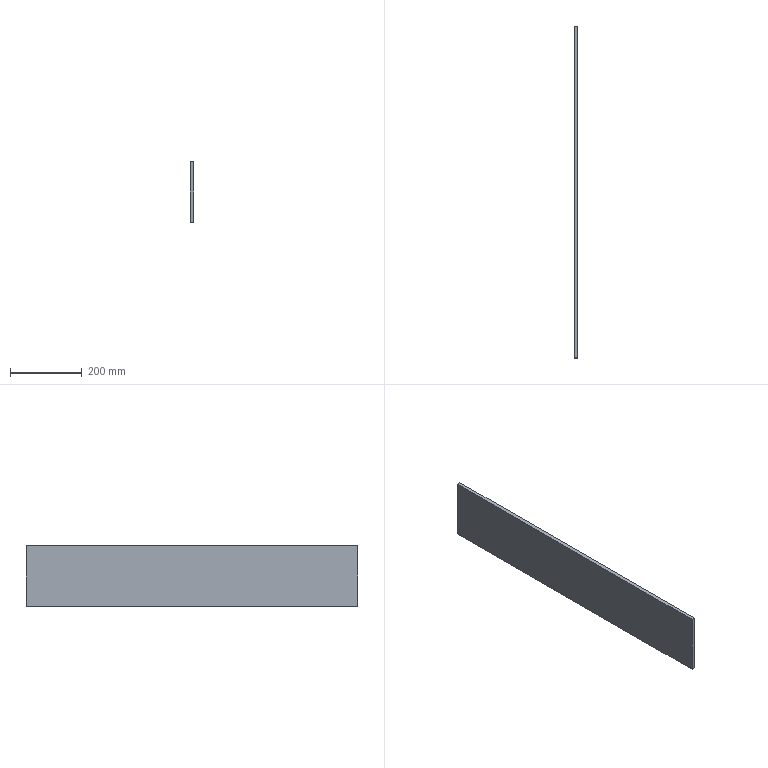Component | SolidWorks | SolderBoxFixingBracketOne-2 | 1 solid | 6 faces | box 10 x 925 x 170 mm | volume 1572500 mm3 | plane 6 | material Plain Carbon Steel
build123d program:
from build123d import *

# Parameters (mm, degrees)
SKETCH1_W           = 925
SKETCH1_H           = 170
BOSS_EXTRUDE1_DEPTH = 10


with BuildPart() as part:
    # Sketch1 → Boss-Extrude1 (new body)
    with BuildSketch(Plane.XY):
        Rectangle(SKETCH1_W, SKETCH1_H)
    extrude(amount=BOSS_EXTRUDE1_DEPTH)


solid = part.part

# Placed as in the assembly
solid = solid.moved(Location((-762.135, 81.593, 1078.102), (90, -90, 0)))
STEP:
#1=COLOUR_RGB('',0.7922,0.8196,0.9333);
#2=FILL_AREA_STYLE_COLOUR('',#1);
#3=FILL_AREA_STYLE('',(#2));
#4=SURFACE_STYLE_FILL_AREA(#3);
#5=SURFACE_SIDE_STYLE('',(#4));
#6=SURFACE_STYLE_USAGE(.BOTH.,#5);
#7=PRESENTATION_STYLE_ASSIGNMENT((#6));
#8=CARTESIAN_POINT('',(-30.399,-14.996,45.791));
#9=VERTEX_POINT('',#8);
#10=CARTESIAN_POINT('',(-30.399,-14.996,39.099));
#11=VERTEX_POINT('',#10);
#12=CARTESIAN_POINT('',(-30.399,-14.996,39.099));
#13=DIRECTION('',(-0.,0.,-1.));
#14=VECTOR('',#13,39.37);
#15=LINE('',#12,#14);
#16=EDGE_CURVE('',#9,#11,#15,.T.);
#17=ORIENTED_EDGE('',*,*,#16,.T.);
#18=CARTESIAN_POINT('',(-30.005,-14.996,39.099));
#19=VERTEX_POINT('',#18);
#20=CARTESIAN_POINT('',(-30.005,-14.996,39.099));
#21=DIRECTION('',(-1.,-0.,0.));
#22=VECTOR('',#21,39.37);
#23=LINE('',#20,#22);
#24=EDGE_CURVE('',#19,#11,#23,.T.);
#25=ORIENTED_EDGE('',*,*,#24,.F.);
#26=CARTESIAN_POINT('',(-30.005,-14.996,45.791));
#27=VERTEX_POINT('',#26);
#28=CARTESIAN_POINT('',(-30.005,-14.996,39.099));
#29=DIRECTION('',(-0.,0.,-1.));
#30=VECTOR('',#29,39.37);
#31=LINE('',#28,#30);
#32=EDGE_CURVE('',#27,#19,#31,.T.);
#33=ORIENTED_EDGE('',*,*,#32,.F.);
#34=CARTESIAN_POINT('',(-30.005,-14.996,45.791));
#35=DIRECTION('',(-1.,-0.,0.));
#36=VECTOR('',#35,39.37);
#37=LINE('',#34,#36);
#38=EDGE_CURVE('',#27,#9,#37,.T.);
#39=ORIENTED_EDGE('',*,*,#38,.T.);
#40=EDGE_LOOP('',(#17,#25,#33,#39));
#41=FACE_OUTER_BOUND('',#40,.T.);
#42=CARTESIAN_POINT('',(-30.005,-14.996,39.099));
#43=DIRECTION('',(-0.,1.,0.));
#44=DIRECTION('',(-1.,-0.,0.));
#45=AXIS2_PLACEMENT_3D('',#42,#43,#44);
#46=PLANE('',#45);
#47=ADVANCED_FACE('',(#41),#46,.F.);
#48=CARTESIAN_POINT('',(-30.399,21.421,39.099));
#49=VERTEX_POINT('',#48);
#50=CARTESIAN_POINT('',(-30.399,21.421,39.099));
#51=DIRECTION('',(-0.,1.,0.));
#52=VECTOR('',#51,39.37);
#53=LINE('',#50,#52);
#54=EDGE_CURVE('',#11,#49,#53,.T.);
#55=ORIENTED_EDGE('',*,*,#54,.T.);
#56=CARTESIAN_POINT('',(-30.005,21.421,39.099));
#57=VERTEX_POINT('',#56);
#58=CARTESIAN_POINT('',(-30.005,21.421,39.099));
#59=DIRECTION('',(-1.,-0.,0.));
#60=VECTOR('',#59,39.37);
#61=LINE('',#58,#60);
#62=EDGE_CURVE('',#57,#49,#61,.T.);
#63=ORIENTED_EDGE('',*,*,#62,.F.);
#64=CARTESIAN_POINT('',(-30.005,21.421,39.099));
#65=DIRECTION('',(-0.,1.,0.));
#66=VECTOR('',#65,39.37);
#67=LINE('',#64,#66);
#68=EDGE_CURVE('',#19,#57,#67,.T.);
#69=ORIENTED_EDGE('',*,*,#68,.F.);
#70=ORIENTED_EDGE('',*,*,#24,.T.);
#71=EDGE_LOOP('',(#55,#63,#69,#70));
#72=FACE_OUTER_BOUND('',#71,.T.);
#73=CARTESIAN_POINT('',(-30.005,21.421,39.099));
#74=DIRECTION('',(0.,-0.,1.));
#75=DIRECTION('',(0.,-1.,-0.));
#76=AXIS2_PLACEMENT_3D('',#73,#74,#75);
#77=PLANE('',#76);
#78=ADVANCED_FACE('',(#72),#77,.F.);
#79=CARTESIAN_POINT('',(-30.399,21.421,45.791));
#80=VERTEX_POINT('',#79);
#81=CARTESIAN_POINT('',(-30.399,21.421,39.099));
#82=DIRECTION('',(0.,-0.,1.));
#83=VECTOR('',#82,39.37);
#84=LINE('',#81,#83);
#85=EDGE_CURVE('',#49,#80,#84,.T.);
#86=ORIENTED_EDGE('',*,*,#85,.T.);
#87=CARTESIAN_POINT('',(-30.005,21.421,45.791));
#88=VERTEX_POINT('',#87);
#89=CARTESIAN_POINT('',(-30.005,21.421,45.791));
#90=DIRECTION('',(-1.,-0.,0.));
#91=VECTOR('',#90,39.37);
#92=LINE('',#89,#91);
#93=EDGE_CURVE('',#88,#80,#92,.T.);
#94=ORIENTED_EDGE('',*,*,#93,.F.);
#95=CARTESIAN_POINT('',(-30.005,21.421,39.099));
#96=DIRECTION('',(0.,-0.,1.));
#97=VECTOR('',#96,39.37);
#98=LINE('',#95,#97);
#99=EDGE_CURVE('',#57,#88,#98,.T.);
#100=ORIENTED_EDGE('',*,*,#99,.F.);
#101=ORIENTED_EDGE('',*,*,#62,.T.);
#102=EDGE_LOOP('',(#86,#94,#100,#101));
#103=FACE_OUTER_BOUND('',#102,.T.);
#104=CARTESIAN_POINT('',(-30.005,21.421,39.099));
#105=DIRECTION('',(0.,-1.,-0.));
#106=DIRECTION('',(1.,0.,-0.));
#107=AXIS2_PLACEMENT_3D('',#104,#105,#106);
#108=PLANE('',#107);
#109=ADVANCED_FACE('',(#103),#108,.F.);
#110=CARTESIAN_POINT('',(-30.399,21.421,45.791));
#111=DIRECTION('',(0.,-1.,-0.));
#112=VECTOR('',#111,39.37);
#113=LINE('',#110,#112);
#114=EDGE_CURVE('',#80,#9,#113,.T.);
#115=ORIENTED_EDGE('',*,*,#114,.T.);
#116=ORIENTED_EDGE('',*,*,#38,.F.);
#117=CARTESIAN_POINT('',(-30.005,21.421,45.791));
#118=DIRECTION('',(0.,-1.,-0.));
#119=VECTOR('',#118,39.37);
#120=LINE('',#117,#119);
#121=EDGE_CURVE('',#88,#27,#120,.T.);
#122=ORIENTED_EDGE('',*,*,#121,.F.);
#123=ORIENTED_EDGE('',*,*,#93,.T.);
#124=EDGE_LOOP('',(#115,#116,#122,#123));
#125=FACE_OUTER_BOUND('',#124,.T.);
#126=CARTESIAN_POINT('',(-30.005,21.421,45.791));
#127=DIRECTION('',(-0.,0.,-1.));
#128=DIRECTION('',(-0.,1.,0.));
#129=AXIS2_PLACEMENT_3D('',#126,#127,#128);
#130=PLANE('',#129);
#131=ADVANCED_FACE('',(#125),#130,.F.);
#132=ORIENTED_EDGE('',*,*,#32,.T.);
#133=ORIENTED_EDGE('',*,*,#68,.T.);
#134=ORIENTED_EDGE('',*,*,#99,.T.);
#135=ORIENTED_EDGE('',*,*,#121,.T.);
#136=EDGE_LOOP('',(#132,#133,#134,#135));
#137=FACE_OUTER_BOUND('',#136,.T.);
#138=CARTESIAN_POINT('',(-30.005,3.212,42.445));
#139=DIRECTION('',(1.,0.,-0.));
#140=DIRECTION('',(-0.,1.,0.));
#141=AXIS2_PLACEMENT_3D('',#138,#139,#140);
#142=PLANE('',#141);
#143=ADVANCED_FACE('',(#137),#142,.T.);
#144=ORIENTED_EDGE('',*,*,#16,.F.);
#145=ORIENTED_EDGE('',*,*,#114,.F.);
#146=ORIENTED_EDGE('',*,*,#85,.F.);
#147=ORIENTED_EDGE('',*,*,#54,.F.);
#148=EDGE_LOOP('',(#144,#145,#146,#147));
#149=FACE_OUTER_BOUND('',#148,.T.);
#150=CARTESIAN_POINT('',(-30.399,3.212,42.445));
#151=DIRECTION('',(1.,0.,-0.));
#152=DIRECTION('',(-0.,1.,0.));
#153=AXIS2_PLACEMENT_3D('',#150,#151,#152);
#154=PLANE('',#153);
#155=ADVANCED_FACE('',(#149),#154,.F.);
#156=CLOSED_SHELL('',(#47,#78,#109,#131,#143,#155));
#157=MANIFOLD_SOLID_BREP('',#156);
#158=STYLED_ITEM('',(#7),#157);
#159=(LENGTH_UNIT()NAMED_UNIT(*)SI_UNIT($,.METRE.));
#160=LENGTH_MEASURE_WITH_UNIT(LENGTH_MEASURE(0.0254),#159);
#161=DIMENSIONAL_EXPONENTS(1.,0.,0.,0.,0.,0.,0.);
#162=(CONVERSION_BASED_UNIT('',#160)LENGTH_UNIT()NAMED_UNIT(#161));
#163=UNCERTAINTY_MEASURE_WITH_UNIT(LENGTH_MEASURE(0.00001),#162,'','');
#164=(NAMED_UNIT(*)PLANE_ANGLE_UNIT()SI_UNIT($,.RADIAN.));
#165=(NAMED_UNIT(*)SI_UNIT($,.STERADIAN.)SOLID_ANGLE_UNIT());
#166=(GEOMETRIC_REPRESENTATION_CONTEXT(3)GLOBAL_UNCERTAINTY_ASSIGNED_CONTEXT((#163))GLOBAL_UNIT_ASSIGNED_CONTEXT((#162,#164,#165))REPRESENTATION_CONTEXT('',''));
#167=MECHANICAL_DESIGN_GEOMETRIC_PRESENTATION_REPRESENTATION('',(#158),#166);
#168=PRESENTATION_LAYER_ASSIGNMENT('','',(#158));
#169=CARTESIAN_POINT('',(0.,0.,0.));
#170=DIRECTION('',(0.,0.,1.));
#171=DIRECTION('',(1.,0.,0.));
#172=AXIS2_PLACEMENT_3D('',#169,#170,#171);
#173=(LENGTH_UNIT()NAMED_UNIT(*)SI_UNIT($,.METRE.));
#174=LENGTH_MEASURE_WITH_UNIT(LENGTH_MEASURE(0.0254),#173);
#175=DIMENSIONAL_EXPONENTS(1.,0.,0.,0.,0.,0.,0.);
#176=(CONVERSION_BASED_UNIT('',#174)LENGTH_UNIT()NAMED_UNIT(#175));
#177=UNCERTAINTY_MEASURE_WITH_UNIT(LENGTH_MEASURE(0.00001),#176,'','');
#178=(NAMED_UNIT(*)PLANE_ANGLE_UNIT()SI_UNIT($,.RADIAN.));
#179=(NAMED_UNIT(*)SI_UNIT($,.STERADIAN.)SOLID_ANGLE_UNIT());
#180=(GEOMETRIC_REPRESENTATION_CONTEXT(3)GLOBAL_UNCERTAINTY_ASSIGNED_CONTEXT((#177))GLOBAL_UNIT_ASSIGNED_CONTEXT((#176,#178,#179))REPRESENTATION_CONTEXT('',''));
#181=ADVANCED_BREP_SHAPE_REPRESENTATION('',(#157,#172),#180);